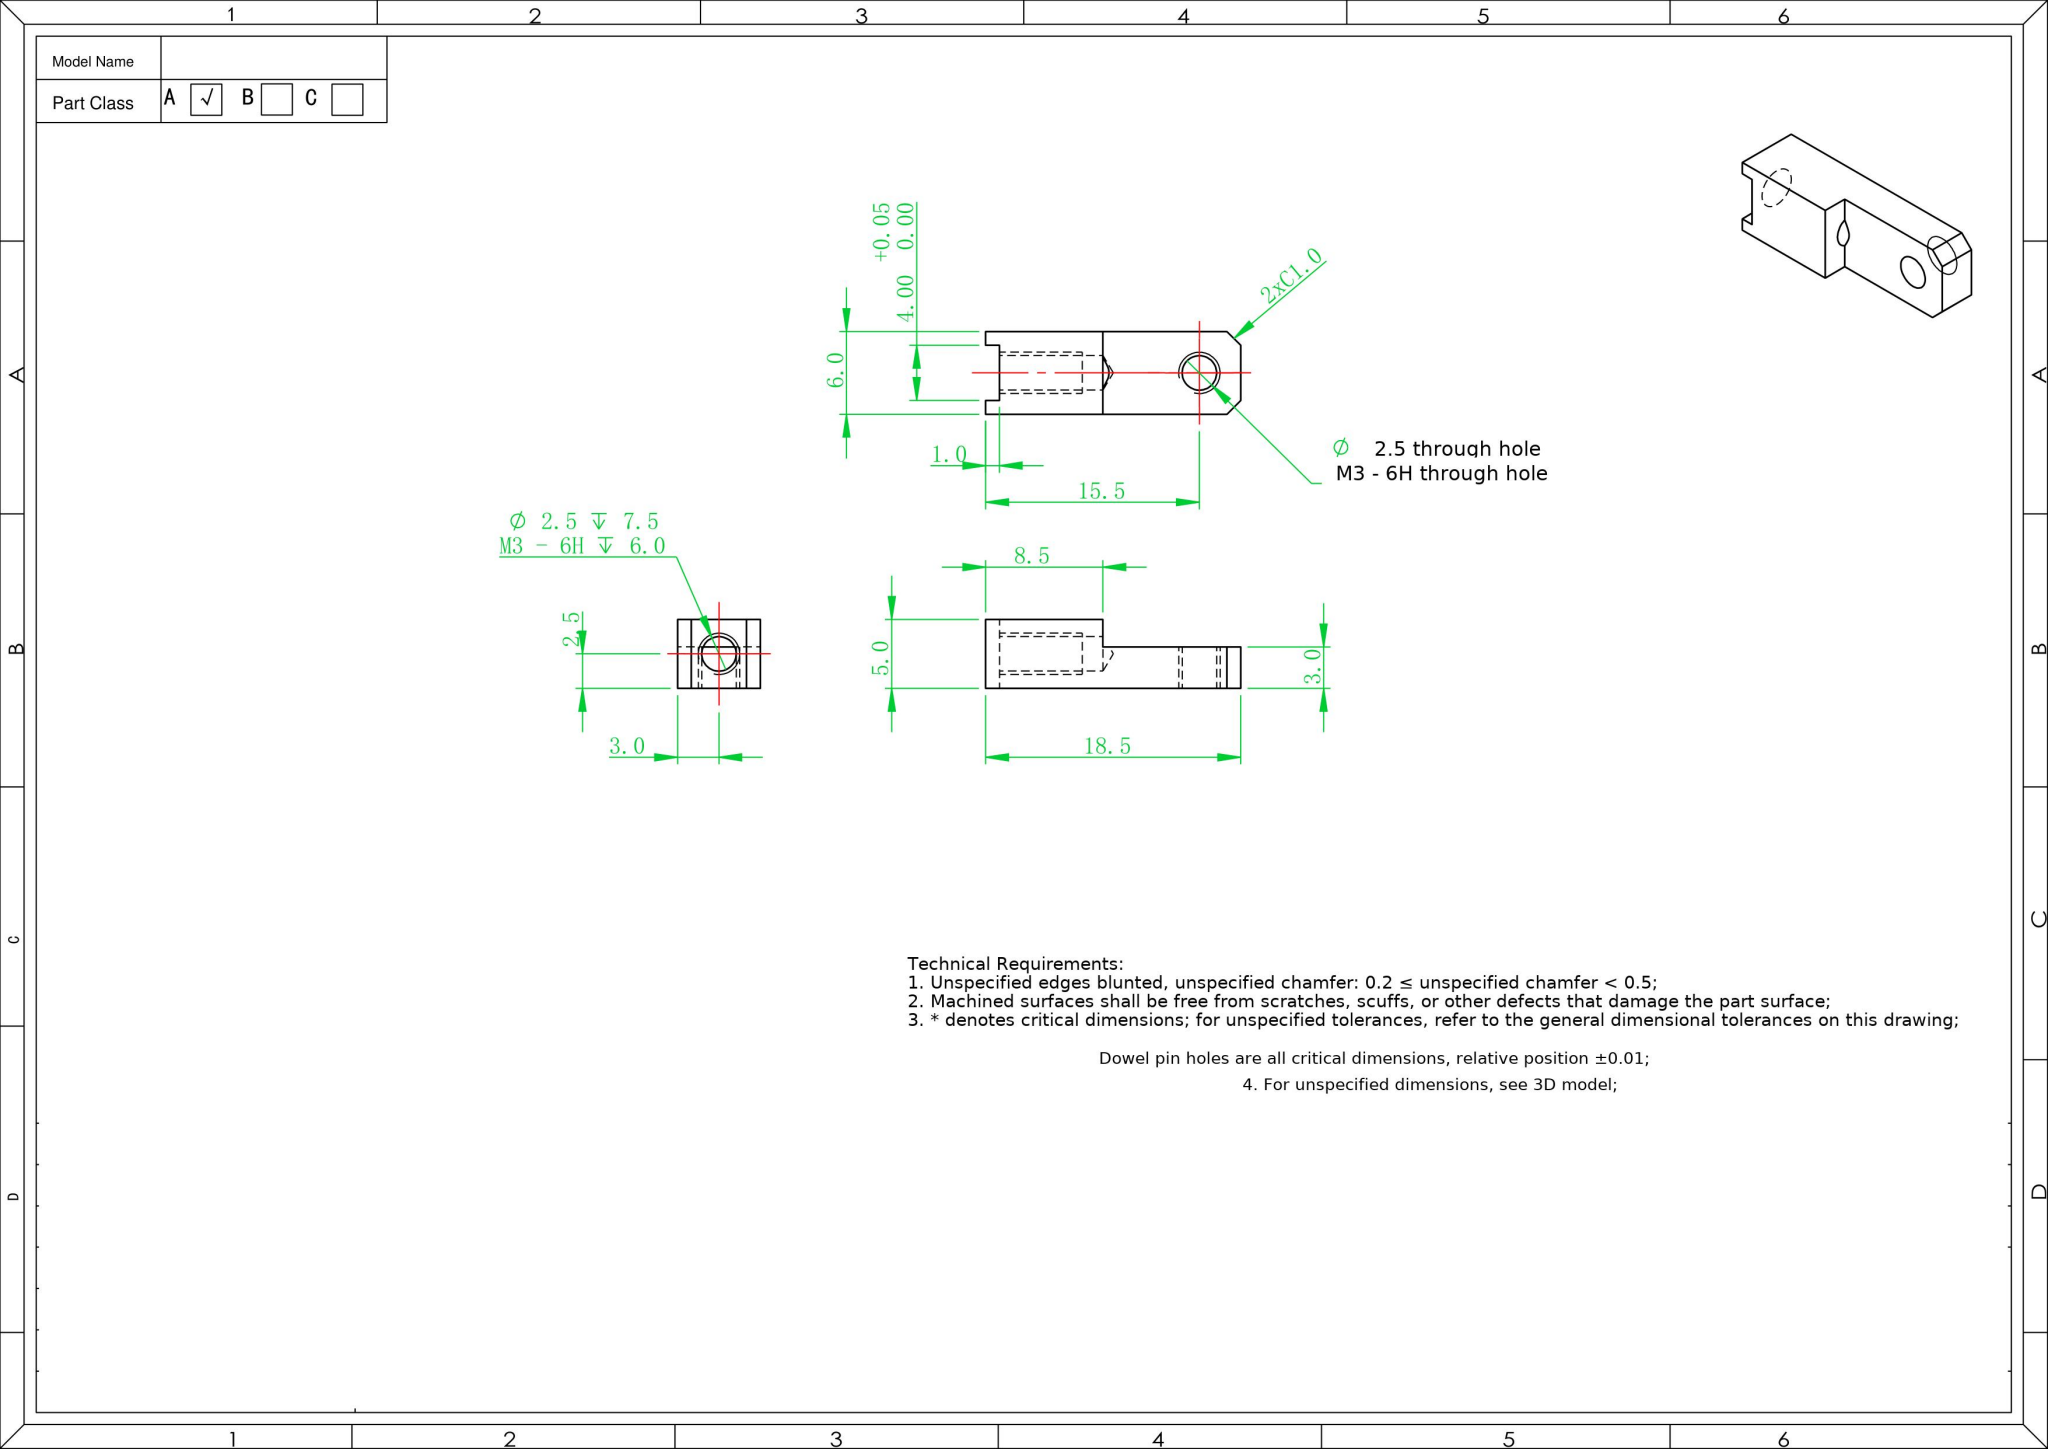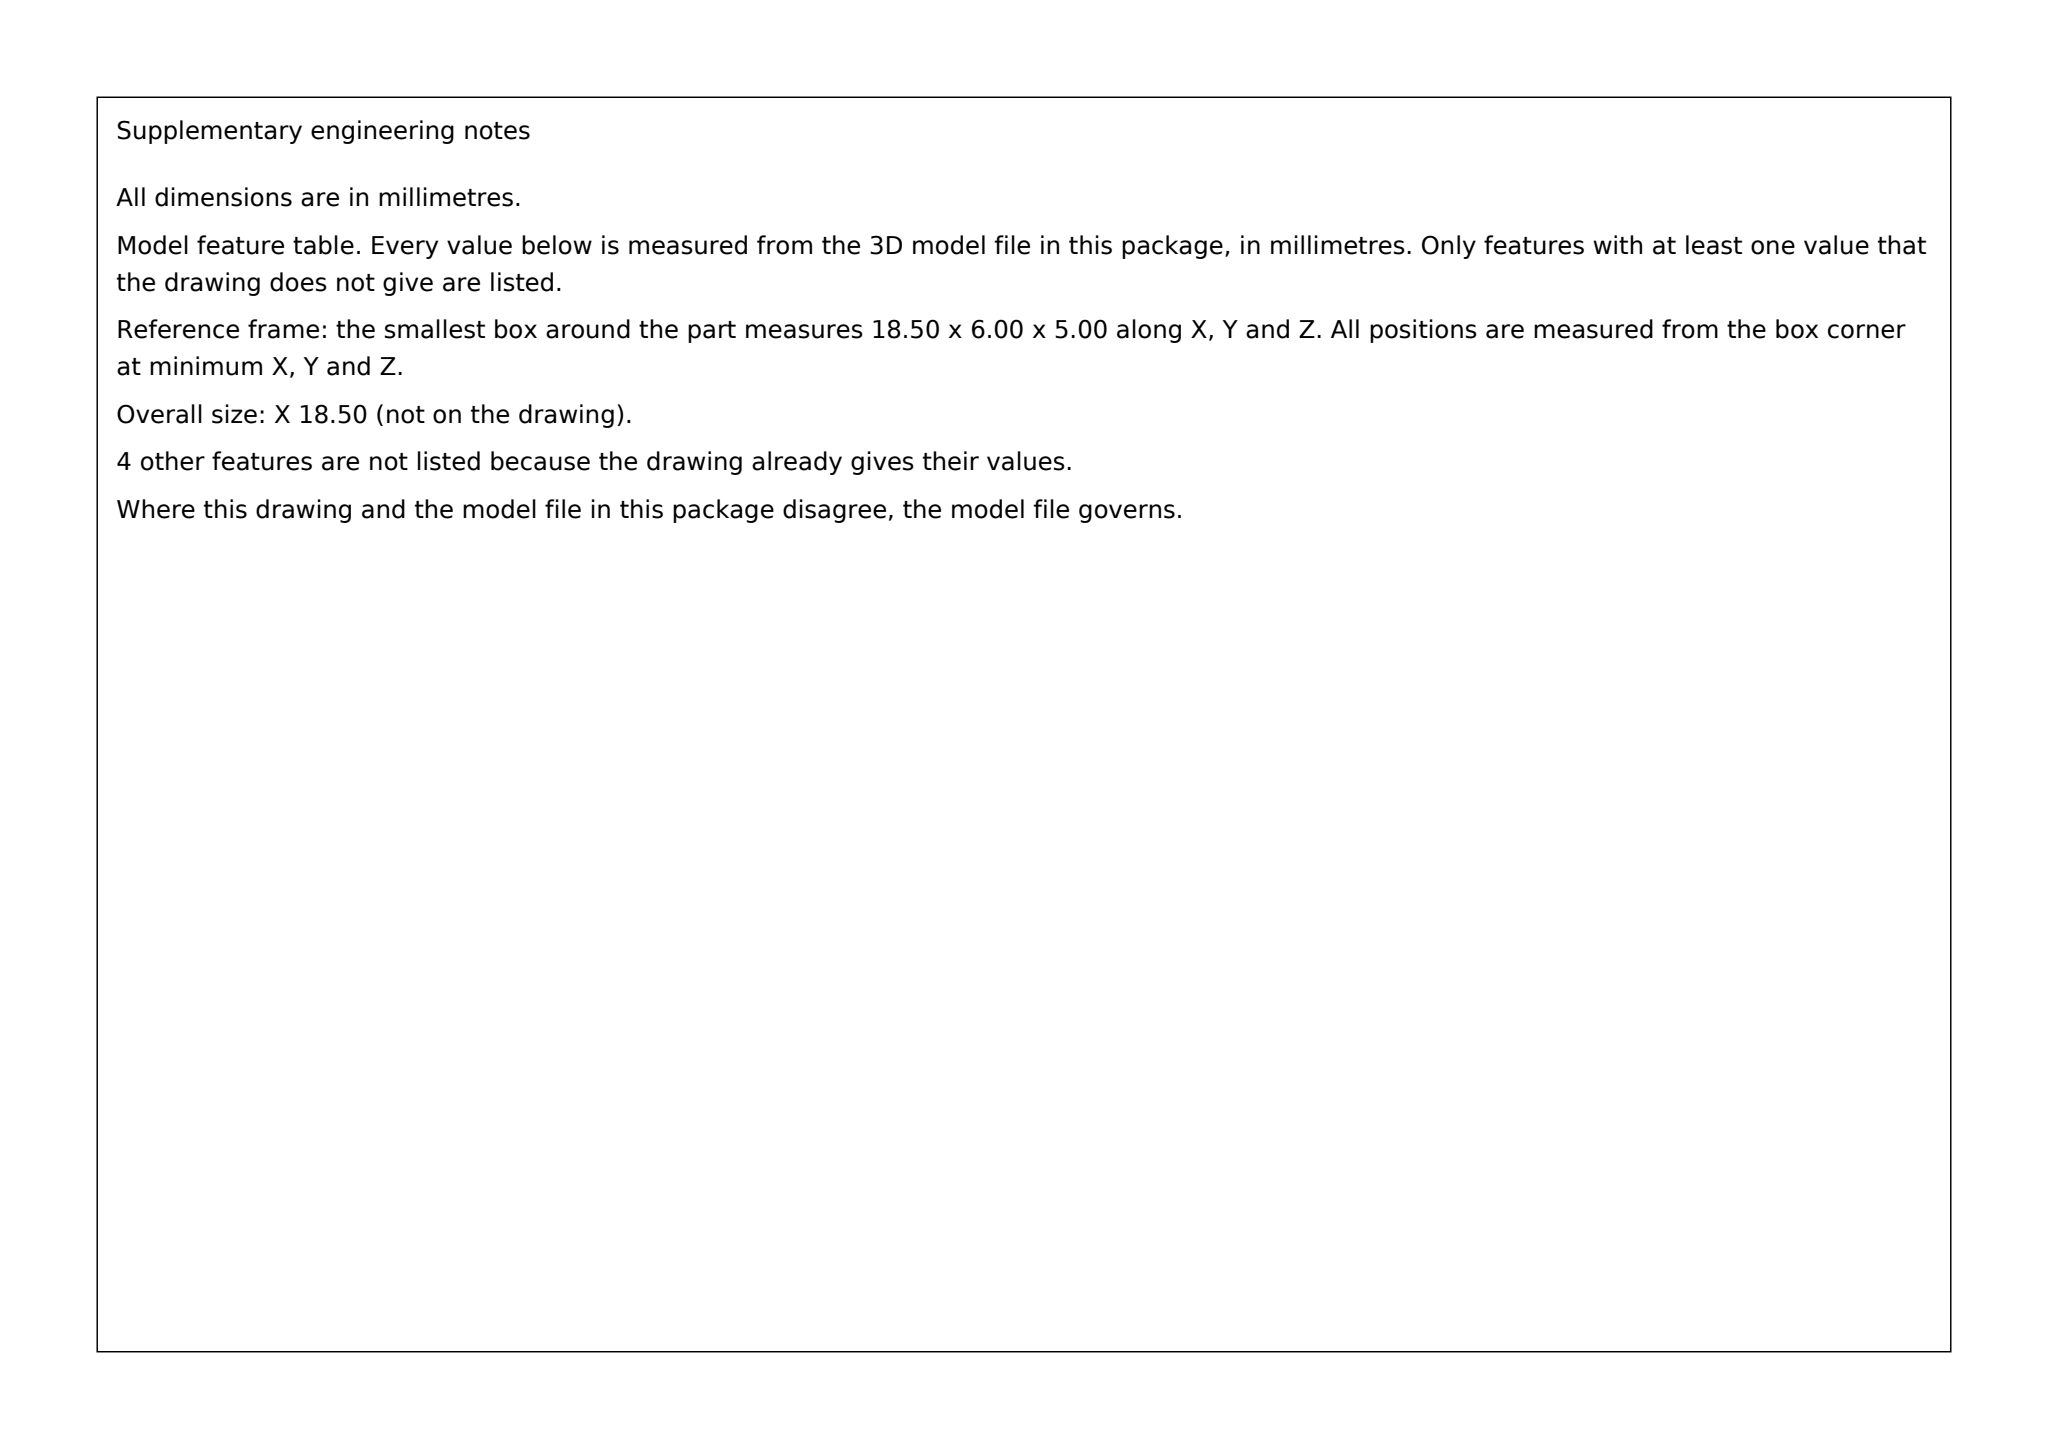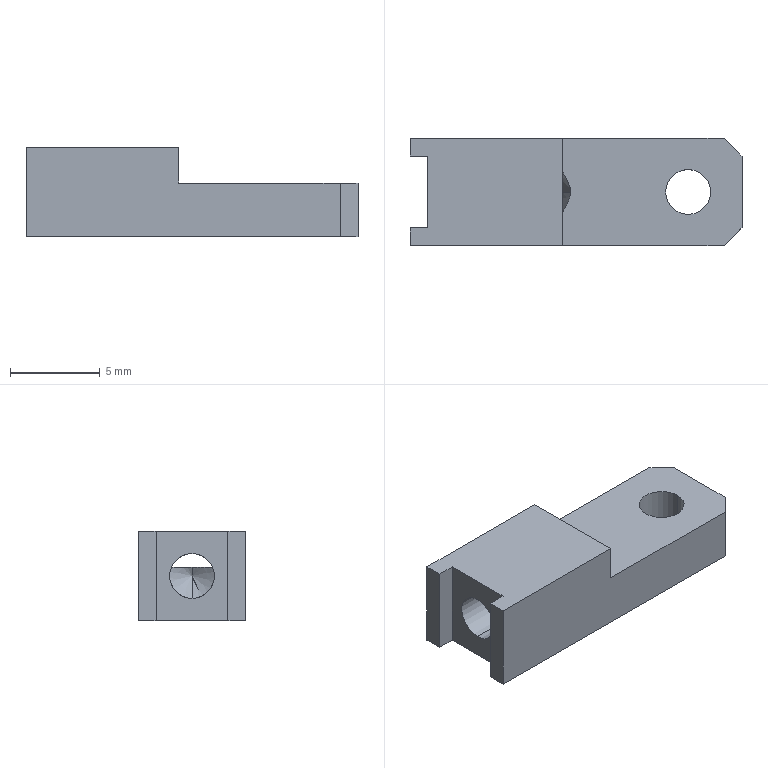Part | SolidWorks | mm | 1 solid | 20 faces | box 18.5 x 6 x 5 mm | volume 359 mm3 | plane 14 | cylinder 4 | cone 2 | commonest cylinder face diameters 2.5 x4
build123d program:
from build123d import *

# Parameters (mm, degrees)
SKETCH1_W             = 17.5
SKETCH1_H             = 6
BOSS_EXTRUDE1_DEPTH   = 5
M3_TAPPED_HOLE1_D     = 2.5
M3_TAPPED_HOLE2_D     = 2.5
M3_TAPPED_HOLE2_DEPTH = 7.5
M3_TAPPED_HOLE2_TIP   = 0.7511
SKETCH6_W             = 5
SKETCH6_H             = 1
BOSS_EXTRUDE2_DEPTH   = 1
SKETCH7_W             = 10
SKETCH7_H             = 2
CUT_EXTRUDE1_DEPTH    = 13.492
CHAMFER1_SIZE         = 1


with BuildPart() as part:
    # Sketch1 → Boss-Extrude1 (new body)
    with BuildSketch(Plane.XY):
        Rectangle(SKETCH1_W, SKETCH1_H)
    extrude(amount=BOSS_EXTRUDE1_DEPTH)

    # M3 Tapped Hole1 (through all)
    with Locations(Plane(origin=(0, 0, 0), x_dir=(-1, 0, 0), z_dir=(0, 0, -1))):
        with Locations((-5.75, 0)):
            Hole(M3_TAPPED_HOLE1_D / 2)

    # M3 Tapped Hole2
    with Locations(Plane.ZY.offset(8.75)):
        with Locations((9.449, -60.488), (2.5, 0)):
            Hole(M3_TAPPED_HOLE2_D / 2, depth=M3_TAPPED_HOLE2_DEPTH)
            with Locations((0, 0, -(M3_TAPPED_HOLE2_DEPTH + M3_TAPPED_HOLE2_TIP / 2))):  # 118° drill point
                Cone(0, M3_TAPPED_HOLE2_D / 2, M3_TAPPED_HOLE2_TIP, mode=Mode.SUBTRACT)

    # Sketch6 → Boss-Extrude2 (add)
    with BuildSketch(Plane.ZY.offset(8.75)):
        with Locations((2.5, 2.5)):
            Rectangle(SKETCH6_W, SKETCH6_H)
        with Locations((2.5, -2.5)):
            Rectangle(SKETCH6_W, SKETCH6_H)
    extrude(amount=BOSS_EXTRUDE2_DEPTH)

    # Sketch7 → Cut-Extrude1 (cut, through all)
    with BuildSketch(Plane.XZ.offset(3)):
        with Locations((3.75, 4)):
            Rectangle(SKETCH7_W, SKETCH7_H)
    extrude(amount=-CUT_EXTRUDE1_DEPTH, mode=Mode.SUBTRACT)

    # Chamfer1
    chamfer1_edges = [part.edges().sort_by_distance(p)[0] for p in [
        (8.75, 3, 1.5),
        (8.75, -3, 1.5),
    ]]
    chamfer(chamfer1_edges, length=CHAMFER1_SIZE)


solid = part.part
STEP:
#1=CARTESIAN_POINT('',(-1.25,0.,1.25));
#2=VERTEX_POINT('',#1);
#3=CARTESIAN_POINT('',(-1.25,-1.146,3.));
#4=VERTEX_POINT('',#3);
#5=CARTESIAN_POINT('',(-1.25,0.,2.5));
#6=DIRECTION('',(-1.,0.,0.));
#7=DIRECTION('',(0.,0.,1.));
#8=AXIS2_PLACEMENT_3D('',#5,#6,#7);
#9=CIRCLE('',#8,1.25);
#10=EDGE_CURVE('',#2,#4,#9,.T.);
#11=ORIENTED_EDGE('',*,*,#10,.F.);
#12=CARTESIAN_POINT('',(-8.75,0.,1.25));
#13=VERTEX_POINT('',#12);
#14=CARTESIAN_POINT('',(-8.75,0.,1.25));
#15=DIRECTION('',(-1.,0.,0.));
#16=VECTOR('',#15,1000.);
#17=LINE('',#14,#16);
#18=EDGE_CURVE('',#2,#13,#17,.T.);
#19=ORIENTED_EDGE('',*,*,#18,.T.);
#20=CARTESIAN_POINT('',(-8.75,0.,3.75));
#21=VERTEX_POINT('',#20);
#22=CARTESIAN_POINT('',(-8.75,0.,2.5));
#23=DIRECTION('',(-1.,0.,0.));
#24=DIRECTION('',(0.,0.,1.));
#25=AXIS2_PLACEMENT_3D('',#22,#23,#24);
#26=CIRCLE('',#25,1.25);
#27=EDGE_CURVE('',#13,#21,#26,.T.);
#28=ORIENTED_EDGE('',*,*,#27,.T.);
#29=CARTESIAN_POINT('',(-1.25,0.,3.75));
#30=VERTEX_POINT('',#29);
#31=CARTESIAN_POINT('',(-8.75,0.,3.75));
#32=DIRECTION('',(-1.,0.,0.));
#33=VECTOR('',#32,1000.);
#34=LINE('',#31,#33);
#35=EDGE_CURVE('',#30,#21,#34,.T.);
#36=ORIENTED_EDGE('',*,*,#35,.F.);
#37=CARTESIAN_POINT('',(-1.25,0.,2.5));
#38=DIRECTION('',(-1.,0.,0.));
#39=DIRECTION('',(0.,0.,1.));
#40=AXIS2_PLACEMENT_3D('',#37,#38,#39);
#41=CIRCLE('',#40,1.25);
#42=EDGE_CURVE('',#4,#30,#41,.T.);
#43=ORIENTED_EDGE('',*,*,#42,.F.);
#44=EDGE_LOOP('',(#11,#19,#28,#36,#43));
#45=FACE_OUTER_BOUND('',#44,.T.);
#46=CARTESIAN_POINT('',(-8.75,0.,2.5));
#47=DIRECTION('',(-1.,0.,0.));
#48=DIRECTION('',(0.,0.,1.));
#49=AXIS2_PLACEMENT_3D('',#46,#47,#48);
#50=CYLINDRICAL_SURFACE('',#49,1.25);
#51=ADVANCED_FACE('',(#45),#50,.F.);
#52=CARTESIAN_POINT('',(-0.4989,0.,2.5));
#53=VERTEX_POINT('',#52);
#54=CARTESIAN_POINT('',(-0.7994,-0.,3.));
#55=VERTEX_POINT('',#54);
#56=CARTESIAN_POINT('',(-1.25,0.,3.75));
#57=DIRECTION('',(-0.515,0.,0.8572));
#58=VECTOR('',#57,1000.);
#59=LINE('',#56,#58);
#60=EDGE_CURVE('',#53,#55,#59,.T.);
#61=ORIENTED_EDGE('',*,*,#60,.F.);
#62=CARTESIAN_POINT('',(-1.25,0.,1.25));
#63=DIRECTION('',(-0.515,0.,-0.8572));
#64=VECTOR('',#63,1000.);
#65=LINE('',#62,#64);
#66=EDGE_CURVE('',#53,#2,#65,.T.);
#67=ORIENTED_EDGE('',*,*,#66,.T.);
#68=ORIENTED_EDGE('',*,*,#10,.T.);
#69=CARTESIAN_POINT('',(-1.25,-1.146,3.));
#70=CARTESIAN_POINT('',(-1.15,-0.9642,3.));
#71=CARTESIAN_POINT('',(-1.052,-0.7817,3.));
#72=CARTESIAN_POINT('',(-0.922,-0.4995,3.));
#73=CARTESIAN_POINT('',(-0.8816,-0.4034,3.));
#74=CARTESIAN_POINT('',(-0.82,-0.2063,3.));
#75=CARTESIAN_POINT('',(-0.7994,-0.1033,3.));
#76=CARTESIAN_POINT('',(-0.7994,-0.,3.));
#77=B_SPLINE_CURVE_WITH_KNOTS('',3,(#69,#70,#71,#72,#73,#74,#75,#76),.UNSPECIFIED.,.F.,.F.,(4,2,2,4),(0.003145,0.003767,0.004078,0.004388),.UNSPECIFIED.);
#78=EDGE_CURVE('',#4,#55,#77,.T.);
#79=ORIENTED_EDGE('',*,*,#78,.T.);
#80=EDGE_LOOP('',(#61,#67,#68,#79));
#81=FACE_OUTER_BOUND('',#80,.T.);
#82=CARTESIAN_POINT('',(-1.25,0.,2.5));
#83=DIRECTION('',(-1.,0.,0.));
#84=DIRECTION('',(0.,0.,1.));
#85=AXIS2_PLACEMENT_3D('',#82,#83,#84);
#86=CONICAL_SURFACE('',#85,1.25,1.03);
#87=ADVANCED_FACE('',(#81),#86,.F.);
#88=CARTESIAN_POINT('',(4.5,0.,3.));
#89=VERTEX_POINT('',#88);
#90=CARTESIAN_POINT('',(7.,0.,3.));
#91=VERTEX_POINT('',#90);
#92=CARTESIAN_POINT('',(5.75,0.,3.));
#93=DIRECTION('',(-0.,-0.,1.));
#94=DIRECTION('',(-1.,0.,0.));
#95=AXIS2_PLACEMENT_3D('',#92,#93,#94);
#96=CIRCLE('',#95,1.25);
#97=EDGE_CURVE('',#89,#91,#96,.T.);
#98=ORIENTED_EDGE('',*,*,#97,.T.);
#99=CARTESIAN_POINT('',(7.,0.,-0.));
#100=VERTEX_POINT('',#99);
#101=CARTESIAN_POINT('',(7.,0.,0.));
#102=DIRECTION('',(0.,0.,-1.));
#103=VECTOR('',#102,1000.);
#104=LINE('',#101,#103);
#105=EDGE_CURVE('',#91,#100,#104,.T.);
#106=ORIENTED_EDGE('',*,*,#105,.T.);
#107=CARTESIAN_POINT('',(4.5,0.,-0.));
#108=VERTEX_POINT('',#107);
#109=CARTESIAN_POINT('',(5.75,0.,-0.));
#110=DIRECTION('',(0.,0.,-1.));
#111=DIRECTION('',(-1.,0.,0.));
#112=AXIS2_PLACEMENT_3D('',#109,#110,#111);
#113=CIRCLE('',#112,1.25);
#114=EDGE_CURVE('',#100,#108,#113,.T.);
#115=ORIENTED_EDGE('',*,*,#114,.T.);
#116=CARTESIAN_POINT('',(4.5,0.,0.));
#117=DIRECTION('',(0.,0.,-1.));
#118=VECTOR('',#117,1000.);
#119=LINE('',#116,#118);
#120=EDGE_CURVE('',#89,#108,#119,.T.);
#121=ORIENTED_EDGE('',*,*,#120,.F.);
#122=EDGE_LOOP('',(#98,#106,#115,#121));
#123=FACE_OUTER_BOUND('',#122,.T.);
#124=CARTESIAN_POINT('',(5.75,0.,0.));
#125=DIRECTION('',(0.,0.,-1.));
#126=DIRECTION('',(-1.,0.,0.));
#127=AXIS2_PLACEMENT_3D('',#124,#125,#126);
#128=CYLINDRICAL_SURFACE('',#127,1.25);
#129=ADVANCED_FACE('',(#123),#128,.F.);
#130=CARTESIAN_POINT('',(-8.75,0.,2.5));
#131=DIRECTION('',(-1.,0.,0.));
#132=DIRECTION('',(0.,0.,1.));
#133=AXIS2_PLACEMENT_3D('',#130,#131,#132);
#134=CIRCLE('',#133,1.25);
#135=EDGE_CURVE('',#21,#13,#134,.T.);
#136=ORIENTED_EDGE('',*,*,#135,.F.);
#137=ORIENTED_EDGE('',*,*,#27,.F.);
#138=EDGE_LOOP('',(#136,#137));
#139=FACE_BOUND('',#138,.T.);
#140=CARTESIAN_POINT('',(-8.75,-2.,5.));
#141=VERTEX_POINT('',#140);
#142=CARTESIAN_POINT('',(-8.75,-2.,0.));
#143=VERTEX_POINT('',#142);
#144=CARTESIAN_POINT('',(-8.75,-2.,5.));
#145=DIRECTION('',(0.,-0.,-1.));
#146=VECTOR('',#145,1000.);
#147=LINE('',#144,#146);
#148=EDGE_CURVE('',#141,#143,#147,.T.);
#149=ORIENTED_EDGE('',*,*,#148,.F.);
#150=CARTESIAN_POINT('',(-8.75,2.,5.));
#151=VERTEX_POINT('',#150);
#152=CARTESIAN_POINT('',(-8.75,3.,5.));
#153=DIRECTION('',(-0.,-1.,0.));
#154=VECTOR('',#153,1000.);
#155=LINE('',#152,#154);
#156=EDGE_CURVE('',#151,#141,#155,.T.);
#157=ORIENTED_EDGE('',*,*,#156,.F.);
#158=CARTESIAN_POINT('',(-8.75,2.,0.));
#159=VERTEX_POINT('',#158);
#160=CARTESIAN_POINT('',(-8.75,2.,5.));
#161=DIRECTION('',(0.,0.,1.));
#162=VECTOR('',#161,1000.);
#163=LINE('',#160,#162);
#164=EDGE_CURVE('',#159,#151,#163,.T.);
#165=ORIENTED_EDGE('',*,*,#164,.F.);
#166=CARTESIAN_POINT('',(-8.75,3.,0.));
#167=DIRECTION('',(-0.,-1.,0.));
#168=VECTOR('',#167,1000.);
#169=LINE('',#166,#168);
#170=EDGE_CURVE('',#159,#143,#169,.T.);
#171=ORIENTED_EDGE('',*,*,#170,.T.);
#172=EDGE_LOOP('',(#149,#157,#165,#171));
#173=FACE_OUTER_BOUND('',#172,.T.);
#174=CARTESIAN_POINT('',(-8.75,3.,5.));
#175=DIRECTION('',(1.,-0.,0.));
#176=DIRECTION('',(0.,1.,0.));
#177=AXIS2_PLACEMENT_3D('',#174,#175,#176);
#178=PLANE('',#177);
#179=ADVANCED_FACE('',(#139,#173),#178,.F.);
#180=CARTESIAN_POINT('',(-9.75,-3.,0.));
#181=VERTEX_POINT('',#180);
#182=CARTESIAN_POINT('',(7.75,-3.,0.));
#183=VERTEX_POINT('',#182);
#184=CARTESIAN_POINT('',(8.75,-3.,0.));
#185=DIRECTION('',(1.,0.,0.));
#186=VECTOR('',#185,1000.);
#187=LINE('',#184,#186);
#188=EDGE_CURVE('',#181,#183,#187,.T.);
#189=ORIENTED_EDGE('',*,*,#188,.T.);
#190=CARTESIAN_POINT('',(7.75,-3.,3.));
#191=VERTEX_POINT('',#190);
#192=CARTESIAN_POINT('',(7.75,-3.,5.));
#193=DIRECTION('',(0.,0.,1.));
#194=VECTOR('',#193,1000.);
#195=LINE('',#192,#194);
#196=EDGE_CURVE('',#183,#191,#195,.T.);
#197=ORIENTED_EDGE('',*,*,#196,.T.);
#198=CARTESIAN_POINT('',(-1.25,-3.,3.));
#199=VERTEX_POINT('',#198);
#200=CARTESIAN_POINT('',(8.75,-3.,3.));
#201=DIRECTION('',(1.,0.,0.));
#202=VECTOR('',#201,1000.);
#203=LINE('',#200,#202);
#204=EDGE_CURVE('',#199,#191,#203,.T.);
#205=ORIENTED_EDGE('',*,*,#204,.F.);
#206=CARTESIAN_POINT('',(-1.25,-3.,5.));
#207=VERTEX_POINT('',#206);
#208=CARTESIAN_POINT('',(-1.25,-3.,5.));
#209=DIRECTION('',(0.,0.,-1.));
#210=VECTOR('',#209,1000.);
#211=LINE('',#208,#210);
#212=EDGE_CURVE('',#207,#199,#211,.T.);
#213=ORIENTED_EDGE('',*,*,#212,.F.);
#214=CARTESIAN_POINT('',(-9.75,-3.,5.));
#215=VERTEX_POINT('',#214);
#216=CARTESIAN_POINT('',(8.75,-3.,5.));
#217=DIRECTION('',(1.,0.,0.));
#218=VECTOR('',#217,1000.);
#219=LINE('',#216,#218);
#220=EDGE_CURVE('',#215,#207,#219,.T.);
#221=ORIENTED_EDGE('',*,*,#220,.F.);
#222=CARTESIAN_POINT('',(-9.75,-3.,5.));
#223=DIRECTION('',(0.,0.,1.));
#224=VECTOR('',#223,1000.);
#225=LINE('',#222,#224);
#226=EDGE_CURVE('',#181,#215,#225,.T.);
#227=ORIENTED_EDGE('',*,*,#226,.F.);
#228=EDGE_LOOP('',(#189,#197,#205,#213,#221,#227));
#229=FACE_OUTER_BOUND('',#228,.T.);
#230=CARTESIAN_POINT('',(8.75,-3.,5.));
#231=DIRECTION('',(-0.,1.,0.));
#232=DIRECTION('',(-1.,-0.,0.));
#233=AXIS2_PLACEMENT_3D('',#230,#231,#232);
#234=PLANE('',#233);
#235=ADVANCED_FACE('',(#229),#234,.F.);
#236=CARTESIAN_POINT('',(8.75,-2.,0.));
#237=VERTEX_POINT('',#236);
#238=CARTESIAN_POINT('',(8.75,2.,0.));
#239=VERTEX_POINT('',#238);
#240=CARTESIAN_POINT('',(8.75,3.,0.));
#241=DIRECTION('',(-0.,1.,0.));
#242=VECTOR('',#241,1000.);
#243=LINE('',#240,#242);
#244=EDGE_CURVE('',#237,#239,#243,.T.);
#245=ORIENTED_EDGE('',*,*,#244,.T.);
#246=CARTESIAN_POINT('',(8.75,2.,3.));
#247=VERTEX_POINT('',#246);
#248=CARTESIAN_POINT('',(8.75,2.,5.));
#249=DIRECTION('',(0.,0.,1.));
#250=VECTOR('',#249,1000.);
#251=LINE('',#248,#250);
#252=EDGE_CURVE('',#239,#247,#251,.T.);
#253=ORIENTED_EDGE('',*,*,#252,.T.);
#254=CARTESIAN_POINT('',(8.75,-2.,3.));
#255=VERTEX_POINT('',#254);
#256=CARTESIAN_POINT('',(8.75,3.,3.));
#257=DIRECTION('',(0.,-1.,0.));
#258=VECTOR('',#257,1000.);
#259=LINE('',#256,#258);
#260=EDGE_CURVE('',#247,#255,#259,.T.);
#261=ORIENTED_EDGE('',*,*,#260,.T.);
#262=CARTESIAN_POINT('',(8.75,-2.,5.));
#263=DIRECTION('',(0.,0.,-1.));
#264=VECTOR('',#263,1000.);
#265=LINE('',#262,#264);
#266=EDGE_CURVE('',#255,#237,#265,.T.);
#267=ORIENTED_EDGE('',*,*,#266,.T.);
#268=EDGE_LOOP('',(#245,#253,#261,#267));
#269=FACE_OUTER_BOUND('',#268,.T.);
#270=CARTESIAN_POINT('',(8.75,3.,5.));
#271=DIRECTION('',(-1.,-0.,0.));
#272=DIRECTION('',(0.,-1.,0.));
#273=AXIS2_PLACEMENT_3D('',#270,#271,#272);
#274=PLANE('',#273);
#275=ADVANCED_FACE('',(#269),#274,.F.);
#276=CARTESIAN_POINT('',(-1.25,3.,3.));
#277=VERTEX_POINT('',#276);
#278=CARTESIAN_POINT('',(7.75,3.,3.));
#279=VERTEX_POINT('',#278);
#280=CARTESIAN_POINT('',(8.75,3.,3.));
#281=DIRECTION('',(1.,0.,0.));
#282=VECTOR('',#281,1000.);
#283=LINE('',#280,#282);
#284=EDGE_CURVE('',#277,#279,#283,.T.);
#285=ORIENTED_EDGE('',*,*,#284,.T.);
#286=CARTESIAN_POINT('',(7.75,3.,0.));
#287=VERTEX_POINT('',#286);
#288=CARTESIAN_POINT('',(7.75,3.,5.));
#289=DIRECTION('',(0.,0.,-1.));
#290=VECTOR('',#289,1000.);
#291=LINE('',#288,#290);
#292=EDGE_CURVE('',#279,#287,#291,.T.);
#293=ORIENTED_EDGE('',*,*,#292,.T.);
#294=CARTESIAN_POINT('',(-9.75,3.,0.));
#295=VERTEX_POINT('',#294);
#296=CARTESIAN_POINT('',(8.75,3.,0.));
#297=DIRECTION('',(-1.,-0.,0.));
#298=VECTOR('',#297,1000.);
#299=LINE('',#296,#298);
#300=EDGE_CURVE('',#287,#295,#299,.T.);
#301=ORIENTED_EDGE('',*,*,#300,.T.);
#302=CARTESIAN_POINT('',(-9.75,3.,5.));
#303=VERTEX_POINT('',#302);
#304=CARTESIAN_POINT('',(-9.75,3.,5.));
#305=DIRECTION('',(0.,0.,-1.));
#306=VECTOR('',#305,1000.);
#307=LINE('',#304,#306);
#308=EDGE_CURVE('',#303,#295,#307,.T.);
#309=ORIENTED_EDGE('',*,*,#308,.F.);
#310=CARTESIAN_POINT('',(-1.25,3.,5.));
#311=VERTEX_POINT('',#310);
#312=CARTESIAN_POINT('',(8.75,3.,5.));
#313=DIRECTION('',(-1.,-0.,0.));
#314=VECTOR('',#313,1000.);
#315=LINE('',#312,#314);
#316=EDGE_CURVE('',#311,#303,#315,.T.);
#317=ORIENTED_EDGE('',*,*,#316,.F.);
#318=CARTESIAN_POINT('',(-1.25,3.,5.));
#319=DIRECTION('',(0.,0.,-1.));
#320=VECTOR('',#319,1000.);
#321=LINE('',#318,#320);
#322=EDGE_CURVE('',#311,#277,#321,.T.);
#323=ORIENTED_EDGE('',*,*,#322,.T.);
#324=EDGE_LOOP('',(#285,#293,#301,#309,#317,#323));
#325=FACE_OUTER_BOUND('',#324,.T.);
#326=CARTESIAN_POINT('',(8.75,3.,5.));
#327=DIRECTION('',(0.,-1.,0.));
#328=DIRECTION('',(1.,0.,0.));
#329=AXIS2_PLACEMENT_3D('',#326,#327,#328);
#330=PLANE('',#329);
#331=ADVANCED_FACE('',(#325),#330,.F.);
#332=ORIENTED_EDGE('',*,*,#220,.T.);
#333=CARTESIAN_POINT('',(-1.25,3.,5.));
#334=DIRECTION('',(0.,-1.,0.));
#335=VECTOR('',#334,1000.);
#336=LINE('',#333,#335);
#337=EDGE_CURVE('',#311,#207,#336,.T.);
#338=ORIENTED_EDGE('',*,*,#337,.F.);
#339=ORIENTED_EDGE('',*,*,#316,.T.);
#340=CARTESIAN_POINT('',(-9.75,2.,5.));
#341=VERTEX_POINT('',#340);
#342=CARTESIAN_POINT('',(-9.75,3.,5.));
#343=DIRECTION('',(-0.,1.,0.));
#344=VECTOR('',#343,1000.);
#345=LINE('',#342,#344);
#346=EDGE_CURVE('',#341,#303,#345,.T.);
#347=ORIENTED_EDGE('',*,*,#346,.F.);
#348=CARTESIAN_POINT('',(-9.75,2.,5.));
#349=DIRECTION('',(1.,0.,0.));
#350=VECTOR('',#349,1000.);
#351=LINE('',#348,#350);
#352=EDGE_CURVE('',#341,#151,#351,.T.);
#353=ORIENTED_EDGE('',*,*,#352,.T.);
#354=ORIENTED_EDGE('',*,*,#156,.T.);
#355=CARTESIAN_POINT('',(-9.75,-2.,5.));
#356=VERTEX_POINT('',#355);
#357=CARTESIAN_POINT('',(-9.75,-2.,5.));
#358=DIRECTION('',(1.,0.,0.));
#359=VECTOR('',#358,1000.);
#360=LINE('',#357,#359);
#361=EDGE_CURVE('',#356,#141,#360,.T.);
#362=ORIENTED_EDGE('',*,*,#361,.F.);
#363=CARTESIAN_POINT('',(-9.75,-3.,5.));
#364=DIRECTION('',(0.,1.,0.));
#365=VECTOR('',#364,1000.);
#366=LINE('',#363,#365);
#367=EDGE_CURVE('',#215,#356,#366,.T.);
#368=ORIENTED_EDGE('',*,*,#367,.F.);
#369=EDGE_LOOP('',(#332,#338,#339,#347,#353,#354,#362,#368));
#370=FACE_OUTER_BOUND('',#369,.T.);
#371=CARTESIAN_POINT('',(0.,0.,5.));
#372=DIRECTION('',(0.,0.,-1.));
#373=DIRECTION('',(-1.,0.,0.));
#374=AXIS2_PLACEMENT_3D('',#371,#372,#373);
#375=PLANE('',#374);
#376=ADVANCED_FACE('',(#370),#375,.F.);
#377=CARTESIAN_POINT('',(5.75,0.,-0.));
#378=DIRECTION('',(0.,0.,-1.));
#379=DIRECTION('',(-1.,0.,0.));
#380=AXIS2_PLACEMENT_3D('',#377,#378,#379);
#381=CIRCLE('',#380,1.25);
#382=EDGE_CURVE('',#108,#100,#381,.T.);
#383=ORIENTED_EDGE('',*,*,#382,.F.);
#384=ORIENTED_EDGE('',*,*,#114,.F.);
#385=EDGE_LOOP('',(#383,#384));
#386=FACE_BOUND('',#385,.T.);
#387=ORIENTED_EDGE('',*,*,#300,.F.);
#388=CARTESIAN_POINT('',(5.375,5.375,0.));
#389=DIRECTION('',(0.7071,-0.7071,0.));
#390=VECTOR('',#389,1000.);
#391=LINE('',#388,#390);
#392=EDGE_CURVE('',#287,#239,#391,.T.);
#393=ORIENTED_EDGE('',*,*,#392,.T.);
#394=ORIENTED_EDGE('',*,*,#244,.F.);
#395=CARTESIAN_POINT('',(5.375,-5.375,0.));
#396=DIRECTION('',(-0.7071,-0.7071,0.));
#397=VECTOR('',#396,1000.);
#398=LINE('',#395,#397);
#399=EDGE_CURVE('',#237,#183,#398,.T.);
#400=ORIENTED_EDGE('',*,*,#399,.T.);
#401=ORIENTED_EDGE('',*,*,#188,.F.);
#402=CARTESIAN_POINT('',(-9.75,-2.,0.));
#403=VERTEX_POINT('',#402);
#404=CARTESIAN_POINT('',(-9.75,-3.,0.));
#405=DIRECTION('',(0.,-1.,0.));
#406=VECTOR('',#405,1000.);
#407=LINE('',#404,#406);
#408=EDGE_CURVE('',#403,#181,#407,.T.);
#409=ORIENTED_EDGE('',*,*,#408,.F.);
#410=CARTESIAN_POINT('',(-9.75,-2.,0.));
#411=DIRECTION('',(1.,0.,0.));
#412=VECTOR('',#411,1000.);
#413=LINE('',#410,#412);
#414=EDGE_CURVE('',#403,#143,#413,.T.);
#415=ORIENTED_EDGE('',*,*,#414,.T.);
#416=ORIENTED_EDGE('',*,*,#170,.F.);
#417=CARTESIAN_POINT('',(-9.75,2.,0.));
#418=VERTEX_POINT('',#417);
#419=CARTESIAN_POINT('',(-9.75,2.,0.));
#420=DIRECTION('',(1.,0.,0.));
#421=VECTOR('',#420,1000.);
#422=LINE('',#419,#421);
#423=EDGE_CURVE('',#418,#159,#422,.T.);
#424=ORIENTED_EDGE('',*,*,#423,.F.);
#425=CARTESIAN_POINT('',(-9.75,3.,0.));
#426=DIRECTION('',(0.,-1.,0.));
#427=VECTOR('',#426,1000.);
#428=LINE('',#425,#427);
#429=EDGE_CURVE('',#295,#418,#428,.T.);
#430=ORIENTED_EDGE('',*,*,#429,.F.);
#431=EDGE_LOOP('',(#387,#393,#394,#400,#401,#409,#415,#416,#424,#430));
#432=FACE_OUTER_BOUND('',#431,.T.);
#433=CARTESIAN_POINT('',(0.,0.,0.));
#434=DIRECTION('',(0.,0.,-1.));
#435=DIRECTION('',(-1.,0.,0.));
#436=AXIS2_PLACEMENT_3D('',#433,#434,#435);
#437=PLANE('',#436);
#438=ADVANCED_FACE('',(#386,#432),#437,.T.);
#439=ORIENTED_EDGE('',*,*,#105,.F.);
#440=CARTESIAN_POINT('',(5.75,0.,3.));
#441=DIRECTION('',(-0.,-0.,1.));
#442=DIRECTION('',(-1.,0.,0.));
#443=AXIS2_PLACEMENT_3D('',#440,#441,#442);
#444=CIRCLE('',#443,1.25);
#445=EDGE_CURVE('',#91,#89,#444,.T.);
#446=ORIENTED_EDGE('',*,*,#445,.T.);
#447=ORIENTED_EDGE('',*,*,#120,.T.);
#448=ORIENTED_EDGE('',*,*,#382,.T.);
#449=EDGE_LOOP('',(#439,#446,#447,#448));
#450=FACE_OUTER_BOUND('',#449,.T.);
#451=CARTESIAN_POINT('',(5.75,0.,0.));
#452=DIRECTION('',(0.,0.,-1.));
#453=DIRECTION('',(-1.,0.,0.));
#454=AXIS2_PLACEMENT_3D('',#451,#452,#453);
#455=CYLINDRICAL_SURFACE('',#454,1.25);
#456=ADVANCED_FACE('',(#450),#455,.F.);
#457=ORIENTED_EDGE('',*,*,#66,.F.);
#458=ORIENTED_EDGE('',*,*,#60,.T.);
#459=CARTESIAN_POINT('',(-1.25,1.146,3.));
#460=VERTEX_POINT('',#459);
#461=CARTESIAN_POINT('',(-0.7994,-0.,3.));
#462=CARTESIAN_POINT('',(-0.7994,0.1041,3.));
#463=CARTESIAN_POINT('',(-0.8197,0.2055,3.));
#464=CARTESIAN_POINT('',(-0.8822,0.4051,3.));
#465=CARTESIAN_POINT('',(-0.9225,0.5005,3.));
#466=CARTESIAN_POINT('',(-1.052,0.7823,3.));
#467=CARTESIAN_POINT('',(-1.15,0.9644,3.));
#468=CARTESIAN_POINT('',(-1.25,1.146,3.));
#469=B_SPLINE_CURVE_WITH_KNOTS('',3,(#461,#462,#463,#464,#465,#466,#467,#468),.UNSPECIFIED.,.F.,.F.,(4,2,2,4),(0.004388,0.004701,0.005014,0.005641),.UNSPECIFIED.);
#470=EDGE_CURVE('',#55,#460,#469,.T.);
#471=ORIENTED_EDGE('',*,*,#470,.T.);
#472=CARTESIAN_POINT('',(-1.25,0.,2.5));
#473=DIRECTION('',(-1.,0.,0.));
#474=DIRECTION('',(0.,0.,1.));
#475=AXIS2_PLACEMENT_3D('',#472,#473,#474);
#476=CIRCLE('',#475,1.25);
#477=EDGE_CURVE('',#460,#2,#476,.T.);
#478=ORIENTED_EDGE('',*,*,#477,.T.);
#479=EDGE_LOOP('',(#457,#458,#471,#478));
#480=FACE_OUTER_BOUND('',#479,.T.);
#481=CARTESIAN_POINT('',(-1.25,0.,2.5));
#482=DIRECTION('',(-1.,0.,0.));
#483=DIRECTION('',(0.,0.,1.));
#484=AXIS2_PLACEMENT_3D('',#481,#482,#483);
#485=CONICAL_SURFACE('',#484,1.25,1.03);
#486=ADVANCED_FACE('',(#480),#485,.F.);
#487=ORIENTED_EDGE('',*,*,#18,.F.);
#488=ORIENTED_EDGE('',*,*,#477,.F.);
#489=CARTESIAN_POINT('',(-1.25,0.,2.5));
#490=DIRECTION('',(-1.,0.,0.));
#491=DIRECTION('',(0.,0.,1.));
#492=AXIS2_PLACEMENT_3D('',#489,#490,#491);
#493=CIRCLE('',#492,1.25);
#494=EDGE_CURVE('',#30,#460,#493,.T.);
#495=ORIENTED_EDGE('',*,*,#494,.F.);
#496=ORIENTED_EDGE('',*,*,#35,.T.);
#497=ORIENTED_EDGE('',*,*,#135,.T.);
#498=EDGE_LOOP('',(#487,#488,#495,#496,#497));
#499=FACE_OUTER_BOUND('',#498,.T.);
#500=CARTESIAN_POINT('',(-8.75,0.,2.5));
#501=DIRECTION('',(-1.,0.,0.));
#502=DIRECTION('',(0.,0.,1.));
#503=AXIS2_PLACEMENT_3D('',#500,#501,#502);
#504=CYLINDRICAL_SURFACE('',#503,1.25);
#505=ADVANCED_FACE('',(#499),#504,.F.);
#506=ORIENTED_EDGE('',*,*,#164,.T.);
#507=ORIENTED_EDGE('',*,*,#352,.F.);
#508=CARTESIAN_POINT('',(-9.75,2.,5.));
#509=DIRECTION('',(0.,0.,1.));
#510=VECTOR('',#509,1000.);
#511=LINE('',#508,#510);
#512=EDGE_CURVE('',#418,#341,#511,.T.);
#513=ORIENTED_EDGE('',*,*,#512,.F.);
#514=ORIENTED_EDGE('',*,*,#423,.T.);
#515=EDGE_LOOP('',(#506,#507,#513,#514));
#516=FACE_OUTER_BOUND('',#515,.T.);
#517=CARTESIAN_POINT('',(-9.75,2.,5.));
#518=DIRECTION('',(-0.,1.,-0.));
#519=DIRECTION('',(-1.,-0.,0.));
#520=AXIS2_PLACEMENT_3D('',#517,#518,#519);
#521=PLANE('',#520);
#522=ADVANCED_FACE('',(#516),#521,.F.);
#523=ORIENTED_EDGE('',*,*,#346,.T.);
#524=ORIENTED_EDGE('',*,*,#308,.T.);
#525=ORIENTED_EDGE('',*,*,#429,.T.);
#526=ORIENTED_EDGE('',*,*,#512,.T.);
#527=EDGE_LOOP('',(#523,#524,#525,#526));
#528=FACE_OUTER_BOUND('',#527,.T.);
#529=CARTESIAN_POINT('',(-9.75,-0.,0.));
#530=DIRECTION('',(1.,0.,-0.));
#531=DIRECTION('',(-0.,1.,0.));
#532=AXIS2_PLACEMENT_3D('',#529,#530,#531);
#533=PLANE('',#532);
#534=ADVANCED_FACE('',(#528),#533,.F.);
#535=ORIENTED_EDGE('',*,*,#148,.T.);
#536=ORIENTED_EDGE('',*,*,#414,.F.);
#537=CARTESIAN_POINT('',(-9.75,-2.,5.));
#538=DIRECTION('',(0.,-0.,-1.));
#539=VECTOR('',#538,1000.);
#540=LINE('',#537,#539);
#541=EDGE_CURVE('',#356,#403,#540,.T.);
#542=ORIENTED_EDGE('',*,*,#541,.F.);
#543=ORIENTED_EDGE('',*,*,#361,.T.);
#544=EDGE_LOOP('',(#535,#536,#542,#543));
#545=FACE_OUTER_BOUND('',#544,.T.);
#546=CARTESIAN_POINT('',(-9.75,-2.,5.));
#547=DIRECTION('',(0.,-1.,0.));
#548=DIRECTION('',(1.,0.,0.));
#549=AXIS2_PLACEMENT_3D('',#546,#547,#548);
#550=PLANE('',#549);
#551=ADVANCED_FACE('',(#545),#550,.F.);
#552=ORIENTED_EDGE('',*,*,#367,.T.);
#553=ORIENTED_EDGE('',*,*,#541,.T.);
#554=ORIENTED_EDGE('',*,*,#408,.T.);
#555=ORIENTED_EDGE('',*,*,#226,.T.);
#556=EDGE_LOOP('',(#552,#553,#554,#555));
#557=FACE_OUTER_BOUND('',#556,.T.);
#558=CARTESIAN_POINT('',(-9.75,-0.,0.));
#559=DIRECTION('',(-1.,0.,0.));
#560=DIRECTION('',(0.,0.,1.));
#561=AXIS2_PLACEMENT_3D('',#558,#559,#560);
#562=PLANE('',#561);
#563=ADVANCED_FACE('',(#557),#562,.T.);
#564=ORIENTED_EDGE('',*,*,#260,.F.);
#565=CARTESIAN_POINT('',(7.75,3.,3.));
#566=DIRECTION('',(-0.7071,0.7071,-0.));
#567=VECTOR('',#566,1000.);
#568=LINE('',#565,#567);
#569=EDGE_CURVE('',#247,#279,#568,.T.);
#570=ORIENTED_EDGE('',*,*,#569,.T.);
#571=ORIENTED_EDGE('',*,*,#284,.F.);
#572=CARTESIAN_POINT('',(-1.25,3.,3.));
#573=DIRECTION('',(0.,-1.,0.));
#574=VECTOR('',#573,1000.);
#575=LINE('',#572,#574);
#576=EDGE_CURVE('',#277,#460,#575,.T.);
#577=ORIENTED_EDGE('',*,*,#576,.T.);
#578=ORIENTED_EDGE('',*,*,#470,.F.);
#579=ORIENTED_EDGE('',*,*,#78,.F.);
#580=CARTESIAN_POINT('',(-1.25,3.,3.));
#581=DIRECTION('',(0.,-1.,0.));
#582=VECTOR('',#581,1000.);
#583=LINE('',#580,#582);
#584=EDGE_CURVE('',#4,#199,#583,.T.);
#585=ORIENTED_EDGE('',*,*,#584,.T.);
#586=ORIENTED_EDGE('',*,*,#204,.T.);
#587=CARTESIAN_POINT('',(8.75,-2.,3.));
#588=DIRECTION('',(0.7071,0.7071,0.));
#589=VECTOR('',#588,1000.);
#590=LINE('',#587,#589);
#591=EDGE_CURVE('',#191,#255,#590,.T.);
#592=ORIENTED_EDGE('',*,*,#591,.T.);
#593=EDGE_LOOP('',(#564,#570,#571,#577,#578,#579,#585,#586,#592));
#594=FACE_OUTER_BOUND('',#593,.T.);
#595=ORIENTED_EDGE('',*,*,#97,.F.);
#596=ORIENTED_EDGE('',*,*,#445,.F.);
#597=EDGE_LOOP('',(#595,#596));
#598=FACE_BOUND('',#597,.T.);
#599=CARTESIAN_POINT('',(8.75,3.,3.));
#600=DIRECTION('',(0.,0.,-1.));
#601=DIRECTION('',(-1.,0.,-0.));
#602=AXIS2_PLACEMENT_3D('',#599,#600,#601);
#603=PLANE('',#602);
#604=ADVANCED_FACE('',(#594,#598),#603,.F.);
#605=ORIENTED_EDGE('',*,*,#576,.F.);
#606=ORIENTED_EDGE('',*,*,#322,.F.);
#607=ORIENTED_EDGE('',*,*,#337,.T.);
#608=ORIENTED_EDGE('',*,*,#212,.T.);
#609=ORIENTED_EDGE('',*,*,#584,.F.);
#610=ORIENTED_EDGE('',*,*,#42,.T.);
#611=ORIENTED_EDGE('',*,*,#494,.T.);
#612=EDGE_LOOP('',(#605,#606,#607,#608,#609,#610,#611));
#613=FACE_OUTER_BOUND('',#612,.T.);
#614=CARTESIAN_POINT('',(-1.25,3.,5.));
#615=DIRECTION('',(-1.,-0.,0.));
#616=DIRECTION('',(0.,-1.,0.));
#617=AXIS2_PLACEMENT_3D('',#614,#615,#616);
#618=PLANE('',#617);
#619=ADVANCED_FACE('',(#613),#618,.F.);
#620=ORIENTED_EDGE('',*,*,#569,.F.);
#621=ORIENTED_EDGE('',*,*,#252,.F.);
#622=ORIENTED_EDGE('',*,*,#392,.F.);
#623=ORIENTED_EDGE('',*,*,#292,.F.);
#624=EDGE_LOOP('',(#620,#621,#622,#623));
#625=FACE_OUTER_BOUND('',#624,.T.);
#626=CARTESIAN_POINT('',(7.75,3.,5.));
#627=DIRECTION('',(-0.7071,-0.7071,0.));
#628=DIRECTION('',(0.,0.,-1.));
#629=AXIS2_PLACEMENT_3D('',#626,#627,#628);
#630=PLANE('',#629);
#631=ADVANCED_FACE('',(#625),#630,.F.);
#632=ORIENTED_EDGE('',*,*,#591,.F.);
#633=ORIENTED_EDGE('',*,*,#196,.F.);
#634=ORIENTED_EDGE('',*,*,#399,.F.);
#635=ORIENTED_EDGE('',*,*,#266,.F.);
#636=EDGE_LOOP('',(#632,#633,#634,#635));
#637=FACE_OUTER_BOUND('',#636,.T.);
#638=CARTESIAN_POINT('',(8.75,-2.,5.));
#639=DIRECTION('',(-0.7071,0.7071,0.));
#640=DIRECTION('',(0.,0.,-1.));
#641=AXIS2_PLACEMENT_3D('',#638,#639,#640);
#642=PLANE('',#641);
#643=ADVANCED_FACE('',(#637),#642,.F.);
#644=CLOSED_SHELL('',(#51,#87,#129,#179,#235,#275,#331,#376,#438,#456,#486,#505,#522,#534,#551,#563,#604,#619,#631,#643));
#645=MANIFOLD_SOLID_BREP('',#644);
#646=CARTESIAN_POINT('',(0.,0.,0.));
#647=DIRECTION('',(0.,0.,1.));
#648=DIRECTION('',(1.,0.,0.));
#649=AXIS2_PLACEMENT_3D('',#646,#647,#648);
#650=(LENGTH_UNIT()NAMED_UNIT(*)SI_UNIT(.MILLI.,.METRE.));
#651=UNCERTAINTY_MEASURE_WITH_UNIT(LENGTH_MEASURE(0.00001),#650,'','');
#652=(NAMED_UNIT(*)PLANE_ANGLE_UNIT()SI_UNIT($,.RADIAN.));
#653=(NAMED_UNIT(*)SI_UNIT($,.STERADIAN.)SOLID_ANGLE_UNIT());
#654=(GEOMETRIC_REPRESENTATION_CONTEXT(3)GLOBAL_UNCERTAINTY_ASSIGNED_CONTEXT((#651))GLOBAL_UNIT_ASSIGNED_CONTEXT((#650,#652,#653))REPRESENTATION_CONTEXT('',''));
#655=ADVANCED_BREP_SHAPE_REPRESENTATION('',(#645,#649),#654);